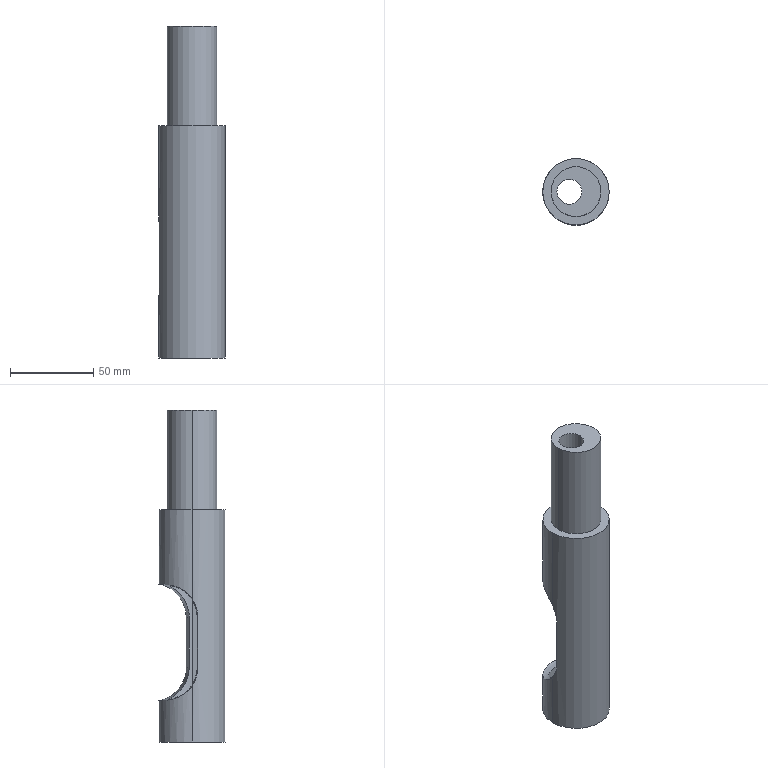Component | SolidWorks | 13EccentricSleeve-1 | 1 solid | 19 faces | box 40 x 40 x 200 mm | volume 119735 mm3 | cylinder 12 | plane 7 | commonest cylinder face diameters 40 x4 15 x2 16 x2 27.5 x2 30 x2
build123d program:
from build123d import *

# Parameters (mm, degrees)
SKETCH1_R               = 20
BOSS_EXTRUDE1_DEPTH     = 140
SKETCH2_R               = 15
BOSS_EXTRUDE2_DEPTH     = 60
SKETCH3_R               = 13.75
CUT_EXTRUDE1_DEPTH      = 100
SKETCH4_R               = 8
CUT_EXTRUDE2_DEPTH      = 80
SKETCH5_R               = 7.5
CUT_EXTRUDE3_DEPTH      = 183.209
CUT_EXTRUDE4_DEPTH      = 202.99
CUT_EXTRUDE4_DEPTH_BACK = 202.99


with BuildPart() as part:
    # Sketch1 → Boss-Extrude1 (new body)
    with BuildSketch(Plane(origin=(0, 0, 0), x_dir=(0, 0, -1), z_dir=(1, 0, 0))):
        Circle(SKETCH1_R)
    extrude(amount=BOSS_EXTRUDE1_DEPTH)

    # Sketch2 → Boss-Extrude2 (add)
    with BuildSketch(Plane(origin=(140, 0, 0), x_dir=(0, 0, -1), z_dir=(1, 0, 0))):
        Circle(SKETCH2_R)
    extrude(amount=BOSS_EXTRUDE2_DEPTH)

    # Sketch3 → Cut-Extrude1 (cut)
    with BuildSketch(Plane.ZY):
        with Locations((4, 0)):
            Circle(SKETCH3_R)
    extrude(amount=-CUT_EXTRUDE1_DEPTH, mode=Mode.SUBTRACT)

    # Sketch4 → Cut-Extrude2 (cut)
    with BuildSketch(Plane.ZY.offset(-100)):
        with Locations((4, 0)):
            Circle(SKETCH4_R)
    extrude(amount=-CUT_EXTRUDE2_DEPTH, mode=Mode.SUBTRACT)

    # Sketch5 → Cut-Extrude3 (cut, through all)
    with BuildSketch(Plane.ZY.offset(-180)):
        with Locations((4, 0)):
            Circle(SKETCH5_R)
    extrude(amount=-CUT_EXTRUDE3_DEPTH, mode=Mode.SUBTRACT)

    # Sketch8 → Cut-Extrude4 (cut, two sides: drawn at the far end of the back side and taken through both)
    with BuildSketch(Plane(origin=(0, 0, 0), x_dir=(-1, 0, 0), z_dir=(0, 0.1736, -0.9848)).offset(-CUT_EXTRUDE4_DEPTH_BACK)):
        with BuildLine():
            Line((-45, 0), (-75, 0))
            ThreePointArc((-75, 0), (-95, 20), (-75, 40))
            Line((-75, 40), (-45, 40))
            ThreePointArc((-45, 40), (-25, 20), (-45, 0))
        make_face()
    extrude(amount=CUT_EXTRUDE4_DEPTH + CUT_EXTRUDE4_DEPTH_BACK, mode=Mode.SUBTRACT)


solid = part.part

# Placed as in the assembly
solid = solid.moved(Location((37.957, -55.224, 190), (0, -90, 0)))
STEP:
#1=COLOUR_RGB('',0.7922,0.8196,0.9333);
#2=FILL_AREA_STYLE_COLOUR('',#1);
#3=FILL_AREA_STYLE('',(#2));
#4=SURFACE_STYLE_FILL_AREA(#3);
#5=SURFACE_SIDE_STYLE('',(#4));
#6=SURFACE_STYLE_USAGE(.BOTH.,#5);
#7=PRESENTATION_STYLE_ASSIGNMENT((#6));
#8=CARTESIAN_POINT('',(1.632,-2.174,15.354));
#9=VERTEX_POINT('',#8);
#10=CARTESIAN_POINT('',(1.042,-2.174,15.354));
#11=VERTEX_POINT('',#10);
#12=CARTESIAN_POINT('',(1.337,-2.174,15.354));
#13=DIRECTION('',(0.,-0.,-1.));
#14=DIRECTION('',(-1.,0.,0.));
#15=AXIS2_PLACEMENT_3D('',#12,#13,#14);
#16=CIRCLE('',#15,0.2953);
#17=EDGE_CURVE('',#9,#11,#16,.T.);
#18=ORIENTED_EDGE('',*,*,#17,.F.);
#19=CARTESIAN_POINT('',(1.632,-2.174,14.567));
#20=VERTEX_POINT('',#19);
#21=CARTESIAN_POINT('',(1.632,-2.174,15.354));
#22=DIRECTION('',(0.,-0.,-1.));
#23=VECTOR('',#22,39.37);
#24=LINE('',#21,#23);
#25=EDGE_CURVE('',#9,#20,#24,.T.);
#26=ORIENTED_EDGE('',*,*,#25,.T.);
#27=CARTESIAN_POINT('',(1.042,-2.174,14.567));
#28=VERTEX_POINT('',#27);
#29=CARTESIAN_POINT('',(1.337,-2.174,14.567));
#30=DIRECTION('',(0.,-0.,-1.));
#31=DIRECTION('',(-1.,0.,0.));
#32=AXIS2_PLACEMENT_3D('',#29,#30,#31);
#33=CIRCLE('',#32,0.2953);
#34=EDGE_CURVE('',#20,#28,#33,.T.);
#35=ORIENTED_EDGE('',*,*,#34,.T.);
#36=CARTESIAN_POINT('',(1.042,-2.174,15.354));
#37=DIRECTION('',(0.,-0.,-1.));
#38=VECTOR('',#37,39.37);
#39=LINE('',#36,#38);
#40=EDGE_CURVE('',#11,#28,#39,.T.);
#41=ORIENTED_EDGE('',*,*,#40,.F.);
#42=EDGE_LOOP('',(#18,#26,#35,#41));
#43=FACE_OUTER_BOUND('',#42,.T.);
#44=CARTESIAN_POINT('',(1.337,-2.174,15.354));
#45=DIRECTION('',(0.,-0.,-1.));
#46=DIRECTION('',(-1.,0.,0.));
#47=AXIS2_PLACEMENT_3D('',#44,#45,#46);
#48=CYLINDRICAL_SURFACE('',#47,0.2953);
#49=ADVANCED_FACE('',(#43),#48,.F.);
#50=CARTESIAN_POINT('',(1.652,-2.174,14.567));
#51=VERTEX_POINT('',#50);
#52=CARTESIAN_POINT('',(1.022,-2.174,14.567));
#53=VERTEX_POINT('',#52);
#54=CARTESIAN_POINT('',(1.337,-2.174,14.567));
#55=DIRECTION('',(0.,-0.,-1.));
#56=DIRECTION('',(1.,0.,0.));
#57=AXIS2_PLACEMENT_3D('',#54,#55,#56);
#58=CIRCLE('',#57,0.315);
#59=EDGE_CURVE('',#51,#53,#58,.T.);
#60=ORIENTED_EDGE('',*,*,#59,.F.);
#61=CARTESIAN_POINT('',(1.652,-2.174,11.417));
#62=VERTEX_POINT('',#61);
#63=CARTESIAN_POINT('',(1.652,-2.174,16.245));
#64=DIRECTION('',(0.,-0.,-1.));
#65=VECTOR('',#64,39.37);
#66=LINE('',#63,#65);
#67=EDGE_CURVE('',#51,#62,#66,.T.);
#68=ORIENTED_EDGE('',*,*,#67,.T.);
#69=CARTESIAN_POINT('',(1.022,-2.174,11.417));
#70=VERTEX_POINT('',#69);
#71=CARTESIAN_POINT('',(1.337,-2.174,11.417));
#72=DIRECTION('',(0.,-0.,-1.));
#73=DIRECTION('',(-1.,0.,0.));
#74=AXIS2_PLACEMENT_3D('',#71,#72,#73);
#75=CIRCLE('',#74,0.315);
#76=EDGE_CURVE('',#62,#70,#75,.T.);
#77=ORIENTED_EDGE('',*,*,#76,.T.);
#78=CARTESIAN_POINT('',(1.022,-2.174,16.245));
#79=DIRECTION('',(0.,-0.,-1.));
#80=VECTOR('',#79,39.37);
#81=LINE('',#78,#80);
#82=EDGE_CURVE('',#53,#70,#81,.T.);
#83=ORIENTED_EDGE('',*,*,#82,.F.);
#84=EDGE_LOOP('',(#60,#68,#77,#83));
#85=FACE_OUTER_BOUND('',#84,.T.);
#86=CARTESIAN_POINT('',(1.337,-2.174,16.245));
#87=DIRECTION('',(0.,-0.,-1.));
#88=DIRECTION('',(-1.,0.,0.));
#89=AXIS2_PLACEMENT_3D('',#86,#87,#88);
#90=CYLINDRICAL_SURFACE('',#89,0.315);
#91=ADVANCED_FACE('',(#85),#90,.F.);
#92=CARTESIAN_POINT('',(1.878,-2.174,11.417));
#93=VERTEX_POINT('',#92);
#94=CARTESIAN_POINT('',(0.7956,-2.174,11.417));
#95=VERTEX_POINT('',#94);
#96=CARTESIAN_POINT('',(1.337,-2.174,11.417));
#97=DIRECTION('',(0.,-0.,-1.));
#98=DIRECTION('',(-1.,0.,0.));
#99=AXIS2_PLACEMENT_3D('',#96,#97,#98);
#100=CIRCLE('',#99,0.5413);
#101=EDGE_CURVE('',#93,#95,#100,.T.);
#102=ORIENTED_EDGE('',*,*,#101,.F.);
#103=CARTESIAN_POINT('',(1.878,-2.174,7.48));
#104=VERTEX_POINT('',#103);
#105=CARTESIAN_POINT('',(1.878,-2.174,11.417));
#106=DIRECTION('',(0.,-0.,-1.));
#107=VECTOR('',#106,39.37);
#108=LINE('',#105,#107);
#109=EDGE_CURVE('',#93,#104,#108,.T.);
#110=ORIENTED_EDGE('',*,*,#109,.T.);
#111=CARTESIAN_POINT('',(0.7956,-2.174,7.48));
#112=VERTEX_POINT('',#111);
#113=CARTESIAN_POINT('',(1.337,-2.174,7.48));
#114=DIRECTION('',(0.,-0.,-1.));
#115=DIRECTION('',(-1.,0.,0.));
#116=AXIS2_PLACEMENT_3D('',#113,#114,#115);
#117=CIRCLE('',#116,0.5413);
#118=EDGE_CURVE('',#104,#112,#117,.T.);
#119=ORIENTED_EDGE('',*,*,#118,.T.);
#120=CARTESIAN_POINT('',(0.7956,-2.174,8.832));
#121=VERTEX_POINT('',#120);
#122=CARTESIAN_POINT('',(0.7956,-2.174,11.417));
#123=DIRECTION('',(0.,-0.,-1.));
#124=VECTOR('',#123,39.37);
#125=LINE('',#122,#124);
#126=EDGE_CURVE('',#121,#112,#125,.T.);
#127=ORIENTED_EDGE('',*,*,#126,.F.);
#128=CARTESIAN_POINT('',(0.8092,-2.295,9.252));
#129=VERTEX_POINT('',#128);
#130=CARTESIAN_POINT('',(0.7956,-2.174,8.832));
#131=CARTESIAN_POINT('',(0.7956,-2.194,8.863));
#132=CARTESIAN_POINT('',(0.7966,-2.211,8.895));
#133=CARTESIAN_POINT('',(0.7988,-2.234,8.946));
#134=CARTESIAN_POINT('',(0.7997,-2.241,8.963));
#135=CARTESIAN_POINT('',(0.8014,-2.254,8.998));
#136=CARTESIAN_POINT('',(0.8023,-2.259,9.015));
#137=CARTESIAN_POINT('',(0.8049,-2.275,9.068));
#138=CARTESIAN_POINT('',(0.8064,-2.282,9.104));
#139=CARTESIAN_POINT('',(0.8086,-2.292,9.178));
#140=CARTESIAN_POINT('',(0.8092,-2.295,9.215));
#141=CARTESIAN_POINT('',(0.8092,-2.295,9.252));
#142=B_SPLINE_CURVE_WITH_KNOTS('',3,(#130,#131,#132,#133,#134,#135,#136,#137,#138,#139,#140,#141),.UNSPECIFIED.,.F.,.F.,(4,2,2,2,2,4),(0.05482,0.05761,0.059,0.0604,0.06318,0.06597),.UNSPECIFIED.);
#143=EDGE_CURVE('',#121,#129,#142,.T.);
#144=ORIENTED_EDGE('',*,*,#143,.T.);
#145=CARTESIAN_POINT('',(0.8092,-2.295,10.433));
#146=VERTEX_POINT('',#145);
#147=CARTESIAN_POINT('',(0.8092,-2.295,11.417));
#148=DIRECTION('',(-0.,0.,1.));
#149=VECTOR('',#148,39.37);
#150=LINE('',#147,#149);
#151=EDGE_CURVE('',#129,#146,#150,.T.);
#152=ORIENTED_EDGE('',*,*,#151,.T.);
#153=CARTESIAN_POINT('',(0.7956,-2.174,10.853));
#154=VERTEX_POINT('',#153);
#155=CARTESIAN_POINT('',(0.8092,-2.295,10.433));
#156=CARTESIAN_POINT('',(0.8092,-2.295,10.47));
#157=CARTESIAN_POINT('',(0.8086,-2.292,10.507));
#158=CARTESIAN_POINT('',(0.8064,-2.282,10.58));
#159=CARTESIAN_POINT('',(0.8049,-2.275,10.616));
#160=CARTESIAN_POINT('',(0.8015,-2.255,10.687));
#161=CARTESIAN_POINT('',(0.7996,-2.242,10.722));
#162=CARTESIAN_POINT('',(0.7966,-2.211,10.79));
#163=CARTESIAN_POINT('',(0.7956,-2.194,10.822));
#164=CARTESIAN_POINT('',(0.7956,-2.174,10.853));
#165=B_SPLINE_CURVE_WITH_KNOTS('',3,(#155,#156,#157,#158,#159,#160,#161,#162,#163,#164),.UNSPECIFIED.,.F.,.F.,(4,2,2,2,4),(0.,0.002801,0.005603,0.008404,0.01121),.UNSPECIFIED.);
#166=EDGE_CURVE('',#146,#154,#165,.T.);
#167=ORIENTED_EDGE('',*,*,#166,.T.);
#168=CARTESIAN_POINT('',(0.7956,-2.174,11.417));
#169=DIRECTION('',(0.,-0.,-1.));
#170=VECTOR('',#169,39.37);
#171=LINE('',#168,#170);
#172=EDGE_CURVE('',#95,#154,#171,.T.);
#173=ORIENTED_EDGE('',*,*,#172,.F.);
#174=EDGE_LOOP('',(#102,#110,#119,#127,#144,#152,#167,#173));
#175=FACE_OUTER_BOUND('',#174,.T.);
#176=CARTESIAN_POINT('',(1.337,-2.174,11.417));
#177=DIRECTION('',(0.,-0.,-1.));
#178=DIRECTION('',(-1.,0.,0.));
#179=AXIS2_PLACEMENT_3D('',#176,#177,#178);
#180=CYLINDRICAL_SURFACE('',#179,0.5413);
#181=ADVANCED_FACE('',(#175),#180,.F.);
#182=CARTESIAN_POINT('',(2.085,-2.174,15.354));
#183=VERTEX_POINT('',#182);
#184=CARTESIAN_POINT('',(0.9038,-2.174,15.354));
#185=VERTEX_POINT('',#184);
#186=CARTESIAN_POINT('',(1.494,-2.174,15.354));
#187=DIRECTION('',(-0.,0.,1.));
#188=DIRECTION('',(1.,0.,0.));
#189=AXIS2_PLACEMENT_3D('',#186,#187,#188);
#190=CIRCLE('',#189,0.5906);
#191=EDGE_CURVE('',#183,#185,#190,.T.);
#192=ORIENTED_EDGE('',*,*,#191,.F.);
#193=CARTESIAN_POINT('',(2.085,-2.174,12.992));
#194=VERTEX_POINT('',#193);
#195=CARTESIAN_POINT('',(2.085,-2.174,15.354));
#196=DIRECTION('',(0.,-0.,-1.));
#197=VECTOR('',#196,39.37);
#198=LINE('',#195,#197);
#199=EDGE_CURVE('',#183,#194,#198,.T.);
#200=ORIENTED_EDGE('',*,*,#199,.T.);
#201=CARTESIAN_POINT('',(0.9038,-2.174,12.992));
#202=VERTEX_POINT('',#201);
#203=CARTESIAN_POINT('',(1.494,-2.174,12.992));
#204=DIRECTION('',(-0.,0.,1.));
#205=DIRECTION('',(1.,0.,0.));
#206=AXIS2_PLACEMENT_3D('',#203,#204,#205);
#207=CIRCLE('',#206,0.5906);
#208=EDGE_CURVE('',#194,#202,#207,.T.);
#209=ORIENTED_EDGE('',*,*,#208,.T.);
#210=CARTESIAN_POINT('',(0.9038,-2.174,15.354));
#211=DIRECTION('',(0.,-0.,-1.));
#212=VECTOR('',#211,39.37);
#213=LINE('',#210,#212);
#214=EDGE_CURVE('',#185,#202,#213,.T.);
#215=ORIENTED_EDGE('',*,*,#214,.F.);
#216=EDGE_LOOP('',(#192,#200,#209,#215));
#217=FACE_OUTER_BOUND('',#216,.T.);
#218=CARTESIAN_POINT('',(1.494,-2.174,15.354));
#219=DIRECTION('',(0.,-0.,-1.));
#220=DIRECTION('',(-1.,0.,0.));
#221=AXIS2_PLACEMENT_3D('',#218,#219,#220);
#222=CYLINDRICAL_SURFACE('',#221,0.5906);
#223=ADVANCED_FACE('',(#217),#222,.T.);
#224=CARTESIAN_POINT('',(2.282,-2.174,12.992));
#225=VERTEX_POINT('',#224);
#226=CARTESIAN_POINT('',(0.707,-2.174,12.992));
#227=VERTEX_POINT('',#226);
#228=CARTESIAN_POINT('',(1.494,-2.174,12.992));
#229=DIRECTION('',(-0.,0.,1.));
#230=DIRECTION('',(1.,0.,0.));
#231=AXIS2_PLACEMENT_3D('',#228,#229,#230);
#232=CIRCLE('',#231,0.7874);
#233=EDGE_CURVE('',#225,#227,#232,.T.);
#234=ORIENTED_EDGE('',*,*,#233,.F.);
#235=CARTESIAN_POINT('',(2.282,-2.174,7.48));
#236=VERTEX_POINT('',#235);
#237=CARTESIAN_POINT('',(2.282,-2.174,12.992));
#238=DIRECTION('',(0.,-0.,-1.));
#239=VECTOR('',#238,39.37);
#240=LINE('',#237,#239);
#241=EDGE_CURVE('',#225,#236,#240,.T.);
#242=ORIENTED_EDGE('',*,*,#241,.T.);
#243=CARTESIAN_POINT('',(0.707,-2.174,7.48));
#244=VERTEX_POINT('',#243);
#245=CARTESIAN_POINT('',(1.494,-2.174,7.48));
#246=DIRECTION('',(-0.,0.,1.));
#247=DIRECTION('',(1.,0.,0.));
#248=AXIS2_PLACEMENT_3D('',#245,#246,#247);
#249=CIRCLE('',#248,0.7874);
#250=EDGE_CURVE('',#236,#244,#249,.T.);
#251=ORIENTED_EDGE('',*,*,#250,.T.);
#252=CARTESIAN_POINT('',(0.707,-2.174,8.809));
#253=VERTEX_POINT('',#252);
#254=CARTESIAN_POINT('',(0.707,-2.174,12.992));
#255=DIRECTION('',(0.,-0.,-1.));
#256=VECTOR('',#255,39.37);
#257=LINE('',#254,#256);
#258=EDGE_CURVE('',#253,#244,#257,.T.);
#259=ORIENTED_EDGE('',*,*,#258,.F.);
#260=CARTESIAN_POINT('',(2.27,-2.037,9.252));
#261=VERTEX_POINT('',#260);
#262=CARTESIAN_POINT('',(0.707,-2.174,8.809));
#263=CARTESIAN_POINT('',(0.707,-2.166,8.796));
#264=CARTESIAN_POINT('',(0.7071,-2.157,8.784));
#265=CARTESIAN_POINT('',(0.7078,-2.138,8.76));
#266=CARTESIAN_POINT('',(0.7082,-2.128,8.749));
#267=CARTESIAN_POINT('',(0.7104,-2.098,8.715));
#268=CARTESIAN_POINT('',(0.7126,-2.077,8.694));
#269=CARTESIAN_POINT('',(0.7194,-2.033,8.655));
#270=CARTESIAN_POINT('',(0.7239,-2.01,8.636));
#271=CARTESIAN_POINT('',(0.7328,-1.974,8.611));
#272=CARTESIAN_POINT('',(0.7362,-1.961,8.603));
#273=CARTESIAN_POINT('',(0.7436,-1.936,8.588));
#274=CARTESIAN_POINT('',(0.7477,-1.924,8.58));
#275=CARTESIAN_POINT('',(0.7611,-1.886,8.56));
#276=CARTESIAN_POINT('',(0.7715,-1.861,8.548));
#277=CARTESIAN_POINT('',(0.7896,-1.823,8.532));
#278=CARTESIAN_POINT('',(0.796,-1.81,8.527));
#279=CARTESIAN_POINT('',(0.8097,-1.785,8.518));
#280=CARTESIAN_POINT('',(0.817,-1.772,8.514));
#281=CARTESIAN_POINT('',(0.8555,-1.71,8.494));
#282=CARTESIAN_POINT('',(0.892,-1.664,8.485));
#283=CARTESIAN_POINT('',(0.9448,-1.61,8.476));
#284=CARTESIAN_POINT('',(0.9558,-1.6,8.475));
#285=CARTESIAN_POINT('',(0.9781,-1.579,8.473));
#286=CARTESIAN_POINT('',(0.9895,-1.57,8.471));
#287=CARTESIAN_POINT('',(1.025,-1.542,8.469));
#288=CARTESIAN_POINT('',(1.049,-1.524,8.468));
#289=CARTESIAN_POINT('',(1.087,-1.5,8.466));
#290=CARTESIAN_POINT('',(1.1,-1.492,8.466));
#291=CARTESIAN_POINT('',(1.126,-1.478,8.465));
#292=CARTESIAN_POINT('',(1.14,-1.471,8.465));
#293=CARTESIAN_POINT('',(1.181,-1.451,8.465));
#294=CARTESIAN_POINT('',(1.208,-1.44,8.465));
#295=CARTESIAN_POINT('',(1.265,-1.42,8.465));
#296=CARTESIAN_POINT('',(1.294,-1.412,8.465));
#297=CARTESIAN_POINT('',(1.352,-1.399,8.465));
#298=CARTESIAN_POINT('',(1.382,-1.394,8.465));
#299=CARTESIAN_POINT('',(1.472,-1.385,8.465));
#300=CARTESIAN_POINT('',(1.532,-1.385,8.465));
#301=CARTESIAN_POINT('',(1.621,-1.397,8.466));
#302=CARTESIAN_POINT('',(1.651,-1.402,8.466));
#303=CARTESIAN_POINT('',(1.71,-1.416,8.468));
#304=CARTESIAN_POINT('',(1.738,-1.425,8.47));
#305=CARTESIAN_POINT('',(1.794,-1.445,8.474));
#306=CARTESIAN_POINT('',(1.822,-1.457,8.477));
#307=CARTESIAN_POINT('',(1.862,-1.477,8.482));
#308=CARTESIAN_POINT('',(1.875,-1.485,8.484));
#309=CARTESIAN_POINT('',(1.901,-1.5,8.489));
#310=CARTESIAN_POINT('',(1.913,-1.507,8.491));
#311=CARTESIAN_POINT('',(1.975,-1.548,8.505));
#312=CARTESIAN_POINT('',(2.019,-1.584,8.521));
#313=CARTESIAN_POINT('',(2.068,-1.635,8.549));
#314=CARTESIAN_POINT('',(2.078,-1.645,8.555));
#315=CARTESIAN_POINT('',(2.096,-1.665,8.568));
#316=CARTESIAN_POINT('',(2.104,-1.676,8.575));
#317=CARTESIAN_POINT('',(2.129,-1.707,8.597));
#318=CARTESIAN_POINT('',(2.143,-1.727,8.612));
#319=CARTESIAN_POINT('',(2.17,-1.769,8.647));
#320=CARTESIAN_POINT('',(2.182,-1.789,8.667));
#321=CARTESIAN_POINT('',(2.202,-1.828,8.708));
#322=CARTESIAN_POINT('',(2.211,-1.847,8.729));
#323=CARTESIAN_POINT('',(2.222,-1.874,8.764));
#324=CARTESIAN_POINT('',(2.226,-1.882,8.776));
#325=CARTESIAN_POINT('',(2.232,-1.899,8.8));
#326=CARTESIAN_POINT('',(2.235,-1.907,8.812));
#327=CARTESIAN_POINT('',(2.243,-1.931,8.85));
#328=CARTESIAN_POINT('',(2.248,-1.945,8.876));
#329=CARTESIAN_POINT('',(2.255,-1.971,8.93));
#330=CARTESIAN_POINT('',(2.258,-1.982,8.958));
#331=CARTESIAN_POINT('',(2.263,-2.002,9.015));
#332=CARTESIAN_POINT('',(2.265,-2.011,9.044));
#333=CARTESIAN_POINT('',(2.269,-2.031,9.132));
#334=CARTESIAN_POINT('',(2.27,-2.037,9.191));
#335=CARTESIAN_POINT('',(2.27,-2.037,9.252));
#336=B_SPLINE_CURVE_WITH_KNOTS('',3,(#262,#263,#264,#265,#266,#267,#268,#269,#270,#271,#272,#273,#274,#275,#276,#277,#278,#279,#280,#281,#282,#283,#284,#285,#286,#287,#288,#289,#290,#291,#292,#293,#294,#295,#296,#297,#298,#299,#300,#301,#302,#303,#304,#305,#306,#307,#308,#309,#310,#311,#312,#313,#314,#315,#316,#317,#318,#319,#320,#321,#322,#323,#324,#325,#326,#327,#328,#329,#330,#331,#332,#333,#334,#335),.UNSPECIFIED.,.F.,.F.,(4,2,2,2,2,2,2,2,2,2,2,2,2,2,2,2,2,2,2,2,2,2,2,2,2,2,2,2,2,2,2,2,2,2,2,2,4),(0.01193,0.01306,0.0142,0.01648,0.01875,0.01989,0.02103,0.0233,0.02444,0.02558,0.03013,0.03126,0.0324,0.03468,0.03581,0.03695,0.03923,0.0415,0.04378,0.04833,0.0506,0.05288,0.05515,0.05629,0.05743,0.06198,0.06311,0.06425,0.06652,0.0688,0.07107,0.07221,0.07335,0.07562,0.0779,0.08017,0.08472),.UNSPECIFIED.);
#337=EDGE_CURVE('',#253,#261,#336,.T.);
#338=ORIENTED_EDGE('',*,*,#337,.T.);
#339=CARTESIAN_POINT('',(2.27,-2.037,10.433));
#340=VERTEX_POINT('',#339);
#341=CARTESIAN_POINT('',(2.27,-2.037,12.992));
#342=DIRECTION('',(-0.,0.,1.));
#343=VECTOR('',#342,39.37);
#344=LINE('',#341,#343);
#345=EDGE_CURVE('',#261,#340,#344,.T.);
#346=ORIENTED_EDGE('',*,*,#345,.T.);
#347=CARTESIAN_POINT('',(0.707,-2.174,10.876));
#348=VERTEX_POINT('',#347);
#349=CARTESIAN_POINT('',(2.27,-2.037,10.433));
#350=CARTESIAN_POINT('',(2.27,-2.037,10.494));
#351=CARTESIAN_POINT('',(2.269,-2.031,10.553));
#352=CARTESIAN_POINT('',(2.265,-2.011,10.641));
#353=CARTESIAN_POINT('',(2.263,-2.002,10.67));
#354=CARTESIAN_POINT('',(2.258,-1.983,10.727));
#355=CARTESIAN_POINT('',(2.255,-1.971,10.754));
#356=CARTESIAN_POINT('',(2.248,-1.946,10.808));
#357=CARTESIAN_POINT('',(2.244,-1.932,10.834));
#358=CARTESIAN_POINT('',(2.236,-1.908,10.871));
#359=CARTESIAN_POINT('',(2.233,-1.9,10.884));
#360=CARTESIAN_POINT('',(2.226,-1.884,10.908));
#361=CARTESIAN_POINT('',(2.223,-1.875,10.92));
#362=CARTESIAN_POINT('',(2.204,-1.83,10.978));
#363=CARTESIAN_POINT('',(2.184,-1.791,11.018));
#364=CARTESIAN_POINT('',(2.151,-1.74,11.062));
#365=CARTESIAN_POINT('',(2.144,-1.73,11.07));
#366=CARTESIAN_POINT('',(2.13,-1.709,11.087));
#367=CARTESIAN_POINT('',(2.122,-1.698,11.094));
#368=CARTESIAN_POINT('',(2.097,-1.667,11.116));
#369=CARTESIAN_POINT('',(2.08,-1.647,11.129));
#370=CARTESIAN_POINT('',(2.041,-1.607,11.151));
#371=CARTESIAN_POINT('',(2.02,-1.587,11.161));
#372=CARTESIAN_POINT('',(1.987,-1.559,11.174));
#373=CARTESIAN_POINT('',(1.975,-1.55,11.178));
#374=CARTESIAN_POINT('',(1.952,-1.533,11.185));
#375=CARTESIAN_POINT('',(1.94,-1.525,11.188));
#376=CARTESIAN_POINT('',(1.903,-1.5,11.196));
#377=CARTESIAN_POINT('',(1.877,-1.485,11.201));
#378=CARTESIAN_POINT('',(1.837,-1.465,11.206));
#379=CARTESIAN_POINT('',(1.823,-1.459,11.208));
#380=CARTESIAN_POINT('',(1.796,-1.446,11.211));
#381=CARTESIAN_POINT('',(1.782,-1.441,11.212));
#382=CARTESIAN_POINT('',(1.739,-1.425,11.215));
#383=CARTESIAN_POINT('',(1.711,-1.416,11.217));
#384=CARTESIAN_POINT('',(1.667,-1.406,11.218));
#385=CARTESIAN_POINT('',(1.652,-1.403,11.219));
#386=CARTESIAN_POINT('',(1.623,-1.397,11.219));
#387=CARTESIAN_POINT('',(1.608,-1.395,11.219));
#388=CARTESIAN_POINT('',(1.533,-1.385,11.22));
#389=CARTESIAN_POINT('',(1.473,-1.385,11.22));
#390=CARTESIAN_POINT('',(1.398,-1.393,11.22));
#391=CARTESIAN_POINT('',(1.383,-1.395,11.22));
#392=CARTESIAN_POINT('',(1.353,-1.399,11.22));
#393=CARTESIAN_POINT('',(1.338,-1.402,11.22));
#394=CARTESIAN_POINT('',(1.294,-1.412,11.22));
#395=CARTESIAN_POINT('',(1.265,-1.42,11.22));
#396=CARTESIAN_POINT('',(1.209,-1.44,11.22));
#397=CARTESIAN_POINT('',(1.181,-1.451,11.22));
#398=CARTESIAN_POINT('',(1.14,-1.471,11.22));
#399=CARTESIAN_POINT('',(1.127,-1.478,11.22));
#400=CARTESIAN_POINT('',(1.101,-1.492,11.219));
#401=CARTESIAN_POINT('',(1.088,-1.5,11.219));
#402=CARTESIAN_POINT('',(1.024,-1.54,11.217));
#403=CARTESIAN_POINT('',(0.9773,-1.577,11.214));
#404=CARTESIAN_POINT('',(0.9247,-1.63,11.206));
#405=CARTESIAN_POINT('',(0.9145,-1.641,11.204));
#406=CARTESIAN_POINT('',(0.8946,-1.664,11.2));
#407=CARTESIAN_POINT('',(0.885,-1.675,11.197));
#408=CARTESIAN_POINT('',(0.8575,-1.71,11.189));
#409=CARTESIAN_POINT('',(0.8407,-1.734,11.183));
#410=CARTESIAN_POINT('',(0.8103,-1.783,11.168));
#411=CARTESIAN_POINT('',(0.7966,-1.808,11.159));
#412=CARTESIAN_POINT('',(0.7783,-1.846,11.143));
#413=CARTESIAN_POINT('',(0.7725,-1.859,11.138));
#414=CARTESIAN_POINT('',(0.7619,-1.885,11.125));
#415=CARTESIAN_POINT('',(0.757,-1.898,11.119));
#416=CARTESIAN_POINT('',(0.7435,-1.935,11.098));
#417=CARTESIAN_POINT('',(0.7362,-1.96,11.083));
#418=CARTESIAN_POINT('',(0.7272,-1.996,11.058));
#419=CARTESIAN_POINT('',(0.7245,-2.008,11.049));
#420=CARTESIAN_POINT('',(0.7199,-2.032,11.031));
#421=CARTESIAN_POINT('',(0.7178,-2.043,11.021));
#422=CARTESIAN_POINT('',(0.7092,-2.1,10.971));
#423=CARTESIAN_POINT('',(0.707,-2.14,10.926));
#424=CARTESIAN_POINT('',(0.707,-2.174,10.876));
#425=B_SPLINE_CURVE_WITH_KNOTS('',3,(#349,#350,#351,#352,#353,#354,#355,#356,#357,#358,#359,#360,#361,#362,#363,#364,#365,#366,#367,#368,#369,#370,#371,#372,#373,#374,#375,#376,#377,#378,#379,#380,#381,#382,#383,#384,#385,#386,#387,#388,#389,#390,#391,#392,#393,#394,#395,#396,#397,#398,#399,#400,#401,#402,#403,#404,#405,#406,#407,#408,#409,#410,#411,#412,#413,#414,#415,#416,#417,#418,#419,#420,#421,#422,#423,#424),.UNSPECIFIED.,.F.,.F.,(4,2,2,2,2,2,2,2,2,2,2,2,2,2,2,2,2,2,2,2,2,2,2,2,2,2,2,2,2,2,2,2,2,2,2,2,2,4),(0.,0.004553,0.00683,0.009107,0.01138,0.01252,0.01366,0.01821,0.01935,0.02049,0.02277,0.02504,0.02618,0.02732,0.0296,0.03074,0.03187,0.03415,0.03529,0.03643,0.04098,0.04212,0.04326,0.04553,0.04781,0.04895,0.05009,0.05464,0.05578,0.05692,0.05919,0.06147,0.06261,0.06375,0.06603,0.06716,0.0683,0.07286),.UNSPECIFIED.);
#426=EDGE_CURVE('',#340,#348,#425,.T.);
#427=ORIENTED_EDGE('',*,*,#426,.T.);
#428=CARTESIAN_POINT('',(0.707,-2.174,12.992));
#429=DIRECTION('',(0.,-0.,-1.));
#430=VECTOR('',#429,39.37);
#431=LINE('',#428,#430);
#432=EDGE_CURVE('',#227,#348,#431,.T.);
#433=ORIENTED_EDGE('',*,*,#432,.F.);
#434=EDGE_LOOP('',(#234,#242,#251,#259,#338,#346,#427,#433));
#435=FACE_OUTER_BOUND('',#434,.T.);
#436=CARTESIAN_POINT('',(1.494,-2.174,12.992));
#437=DIRECTION('',(0.,-0.,-1.));
#438=DIRECTION('',(-1.,0.,0.));
#439=AXIS2_PLACEMENT_3D('',#436,#437,#438);
#440=CYLINDRICAL_SURFACE('',#439,0.7874);
#441=ADVANCED_FACE('',(#435),#440,.T.);
#442=ORIENTED_EDGE('',*,*,#241,.F.);
#443=CARTESIAN_POINT('',(1.494,-2.174,12.992));
#444=DIRECTION('',(-0.,0.,1.));
#445=DIRECTION('',(1.,0.,0.));
#446=AXIS2_PLACEMENT_3D('',#443,#444,#445);
#447=CIRCLE('',#446,0.7874);
#448=EDGE_CURVE('',#227,#225,#447,.T.);
#449=ORIENTED_EDGE('',*,*,#448,.F.);
#450=ORIENTED_EDGE('',*,*,#432,.T.);
#451=CARTESIAN_POINT('',(0.7189,-2.311,10.433));
#452=VERTEX_POINT('',#451);
#453=CARTESIAN_POINT('',(0.707,-2.174,10.876));
#454=CARTESIAN_POINT('',(0.707,-2.185,10.86));
#455=CARTESIAN_POINT('',(0.7072,-2.196,10.844));
#456=CARTESIAN_POINT('',(0.708,-2.216,10.81));
#457=CARTESIAN_POINT('',(0.7086,-2.225,10.792));
#458=CARTESIAN_POINT('',(0.7105,-2.25,10.739));
#459=CARTESIAN_POINT('',(0.7121,-2.265,10.703));
#460=CARTESIAN_POINT('',(0.7151,-2.288,10.627));
#461=CARTESIAN_POINT('',(0.7165,-2.296,10.589));
#462=CARTESIAN_POINT('',(0.7184,-2.308,10.512));
#463=CARTESIAN_POINT('',(0.7189,-2.311,10.473));
#464=CARTESIAN_POINT('',(0.7189,-2.311,10.433));
#465=B_SPLINE_CURVE_WITH_KNOTS('',3,(#453,#454,#455,#456,#457,#458,#459,#460,#461,#462,#463,#464),.UNSPECIFIED.,.F.,.F.,(4,2,2,2,2,4),(0.07286,0.07434,0.07582,0.07879,0.08176,0.08472),.UNSPECIFIED.);
#466=EDGE_CURVE('',#348,#452,#465,.T.);
#467=ORIENTED_EDGE('',*,*,#466,.T.);
#468=CARTESIAN_POINT('',(0.7189,-2.311,9.252));
#469=VERTEX_POINT('',#468);
#470=CARTESIAN_POINT('',(0.7189,-2.311,12.992));
#471=DIRECTION('',(0.,-0.,-1.));
#472=VECTOR('',#471,39.37);
#473=LINE('',#470,#472);
#474=EDGE_CURVE('',#452,#469,#473,.T.);
#475=ORIENTED_EDGE('',*,*,#474,.T.);
#476=CARTESIAN_POINT('',(0.7189,-2.311,9.252));
#477=CARTESIAN_POINT('',(0.7189,-2.311,9.212));
#478=CARTESIAN_POINT('',(0.7184,-2.308,9.173));
#479=CARTESIAN_POINT('',(0.7165,-2.296,9.096));
#480=CARTESIAN_POINT('',(0.7151,-2.288,9.058));
#481=CARTESIAN_POINT('',(0.7129,-2.271,9.001));
#482=CARTESIAN_POINT('',(0.7121,-2.264,8.982));
#483=CARTESIAN_POINT('',(0.7106,-2.25,8.945));
#484=CARTESIAN_POINT('',(0.7098,-2.242,8.927));
#485=CARTESIAN_POINT('',(0.7079,-2.216,8.875));
#486=CARTESIAN_POINT('',(0.707,-2.197,8.841));
#487=CARTESIAN_POINT('',(0.707,-2.174,8.809));
#488=B_SPLINE_CURVE_WITH_KNOTS('',3,(#476,#477,#478,#479,#480,#481,#482,#483,#484,#485,#486,#487),.UNSPECIFIED.,.F.,.F.,(4,2,2,2,2,4),(0.,0.002982,0.005963,0.007454,0.008945,0.01193),.UNSPECIFIED.);
#489=EDGE_CURVE('',#469,#253,#488,.T.);
#490=ORIENTED_EDGE('',*,*,#489,.T.);
#491=ORIENTED_EDGE('',*,*,#258,.T.);
#492=CARTESIAN_POINT('',(1.494,-2.174,7.48));
#493=DIRECTION('',(-0.,0.,1.));
#494=DIRECTION('',(1.,0.,0.));
#495=AXIS2_PLACEMENT_3D('',#492,#493,#494);
#496=CIRCLE('',#495,0.7874);
#497=EDGE_CURVE('',#244,#236,#496,.T.);
#498=ORIENTED_EDGE('',*,*,#497,.T.);
#499=EDGE_LOOP('',(#442,#449,#450,#467,#475,#490,#491,#498));
#500=FACE_OUTER_BOUND('',#499,.T.);
#501=CARTESIAN_POINT('',(1.494,-2.174,12.992));
#502=DIRECTION('',(0.,-0.,-1.));
#503=DIRECTION('',(-1.,0.,0.));
#504=AXIS2_PLACEMENT_3D('',#501,#502,#503);
#505=CYLINDRICAL_SURFACE('',#504,0.7874);
#506=ADVANCED_FACE('',(#500),#505,.T.);
#507=CARTESIAN_POINT('',(1.494,-2.174,12.992));
#508=DIRECTION('',(-0.,0.,1.));
#509=DIRECTION('',(1.,0.,0.));
#510=AXIS2_PLACEMENT_3D('',#507,#508,#509);
#511=CIRCLE('',#510,0.5906);
#512=EDGE_CURVE('',#202,#194,#511,.T.);
#513=ORIENTED_EDGE('',*,*,#512,.F.);
#514=ORIENTED_EDGE('',*,*,#208,.F.);
#515=EDGE_LOOP('',(#513,#514));
#516=FACE_BOUND('',#515,.T.);
#517=ORIENTED_EDGE('',*,*,#448,.T.);
#518=ORIENTED_EDGE('',*,*,#233,.T.);
#519=EDGE_LOOP('',(#517,#518));
#520=FACE_OUTER_BOUND('',#519,.T.);
#521=CARTESIAN_POINT('',(1.494,-2.174,12.992));
#522=DIRECTION('',(-0.,0.,1.));
#523=DIRECTION('',(1.,0.,0.));
#524=AXIS2_PLACEMENT_3D('',#521,#522,#523);
#525=PLANE('',#524);
#526=ADVANCED_FACE('',(#516,#520),#525,.T.);
#527=CARTESIAN_POINT('',(1.337,-2.174,7.48));
#528=DIRECTION('',(0.,-0.,-1.));
#529=DIRECTION('',(-1.,0.,0.));
#530=AXIS2_PLACEMENT_3D('',#527,#528,#529);
#531=CIRCLE('',#530,0.5413);
#532=EDGE_CURVE('',#112,#104,#531,.T.);
#533=ORIENTED_EDGE('',*,*,#532,.F.);
#534=ORIENTED_EDGE('',*,*,#118,.F.);
#535=EDGE_LOOP('',(#533,#534));
#536=FACE_BOUND('',#535,.T.);
#537=ORIENTED_EDGE('',*,*,#497,.F.);
#538=ORIENTED_EDGE('',*,*,#250,.F.);
#539=EDGE_LOOP('',(#537,#538));
#540=FACE_OUTER_BOUND('',#539,.T.);
#541=CARTESIAN_POINT('',(1.494,-2.174,7.48));
#542=DIRECTION('',(-0.,0.,1.));
#543=DIRECTION('',(1.,0.,0.));
#544=AXIS2_PLACEMENT_3D('',#541,#542,#543);
#545=PLANE('',#544);
#546=ADVANCED_FACE('',(#536,#540),#545,.F.);
#547=ORIENTED_EDGE('',*,*,#199,.F.);
#548=CARTESIAN_POINT('',(1.494,-2.174,15.354));
#549=DIRECTION('',(-0.,0.,1.));
#550=DIRECTION('',(1.,0.,0.));
#551=AXIS2_PLACEMENT_3D('',#548,#549,#550);
#552=CIRCLE('',#551,0.5906);
#553=EDGE_CURVE('',#185,#183,#552,.T.);
#554=ORIENTED_EDGE('',*,*,#553,.F.);
#555=ORIENTED_EDGE('',*,*,#214,.T.);
#556=ORIENTED_EDGE('',*,*,#512,.T.);
#557=EDGE_LOOP('',(#547,#554,#555,#556));
#558=FACE_OUTER_BOUND('',#557,.T.);
#559=CARTESIAN_POINT('',(1.494,-2.174,15.354));
#560=DIRECTION('',(0.,-0.,-1.));
#561=DIRECTION('',(-1.,0.,0.));
#562=AXIS2_PLACEMENT_3D('',#559,#560,#561);
#563=CYLINDRICAL_SURFACE('',#562,0.5906);
#564=ADVANCED_FACE('',(#558),#563,.T.);
#565=CARTESIAN_POINT('',(1.337,-2.174,15.354));
#566=DIRECTION('',(0.,-0.,-1.));
#567=DIRECTION('',(-1.,0.,0.));
#568=AXIS2_PLACEMENT_3D('',#565,#566,#567);
#569=CIRCLE('',#568,0.2953);
#570=EDGE_CURVE('',#11,#9,#569,.T.);
#571=ORIENTED_EDGE('',*,*,#570,.T.);
#572=ORIENTED_EDGE('',*,*,#17,.T.);
#573=EDGE_LOOP('',(#571,#572));
#574=FACE_BOUND('',#573,.T.);
#575=ORIENTED_EDGE('',*,*,#553,.T.);
#576=ORIENTED_EDGE('',*,*,#191,.T.);
#577=EDGE_LOOP('',(#575,#576));
#578=FACE_OUTER_BOUND('',#577,.T.);
#579=CARTESIAN_POINT('',(1.494,-2.174,15.354));
#580=DIRECTION('',(-0.,0.,1.));
#581=DIRECTION('',(1.,0.,0.));
#582=AXIS2_PLACEMENT_3D('',#579,#580,#581);
#583=PLANE('',#582);
#584=ADVANCED_FACE('',(#574,#578),#583,.T.);
#585=ORIENTED_EDGE('',*,*,#109,.F.);
#586=CARTESIAN_POINT('',(1.337,-2.174,11.417));
#587=DIRECTION('',(0.,-0.,-1.));
#588=DIRECTION('',(-1.,0.,0.));
#589=AXIS2_PLACEMENT_3D('',#586,#587,#588);
#590=CIRCLE('',#589,0.5413);
#591=EDGE_CURVE('',#95,#93,#590,.T.);
#592=ORIENTED_EDGE('',*,*,#591,.F.);
#593=ORIENTED_EDGE('',*,*,#172,.T.);
#594=CARTESIAN_POINT('',(1.874,-2.107,10.433));
#595=VERTEX_POINT('',#594);
#596=CARTESIAN_POINT('',(0.7956,-2.174,10.853));
#597=CARTESIAN_POINT('',(0.7956,-2.162,10.872));
#598=CARTESIAN_POINT('',(0.796,-2.149,10.89));
#599=CARTESIAN_POINT('',(0.798,-2.121,10.926));
#600=CARTESIAN_POINT('',(0.7996,-2.106,10.944));
#601=CARTESIAN_POINT('',(0.8068,-2.06,10.993));
#602=CARTESIAN_POINT('',(0.8147,-2.027,11.022));
#603=CARTESIAN_POINT('',(0.8306,-1.982,11.055));
#604=CARTESIAN_POINT('',(0.8341,-1.973,11.061));
#605=CARTESIAN_POINT('',(0.8415,-1.956,11.073));
#606=CARTESIAN_POINT('',(0.8456,-1.947,11.079));
#607=CARTESIAN_POINT('',(0.8585,-1.92,11.095));
#608=CARTESIAN_POINT('',(0.8683,-1.902,11.105));
#609=CARTESIAN_POINT('',(0.885,-1.876,11.118));
#610=CARTESIAN_POINT('',(0.8908,-1.867,11.123));
#611=CARTESIAN_POINT('',(0.9032,-1.85,11.131));
#612=CARTESIAN_POINT('',(0.9098,-1.841,11.134));
#613=CARTESIAN_POINT('',(0.9303,-1.816,11.145));
#614=CARTESIAN_POINT('',(0.9451,-1.8,11.151));
#615=CARTESIAN_POINT('',(0.9767,-1.769,11.162));
#616=CARTESIAN_POINT('',(0.9936,-1.755,11.166));
#617=CARTESIAN_POINT('',(1.021,-1.735,11.172));
#618=CARTESIAN_POINT('',(1.03,-1.728,11.174));
#619=CARTESIAN_POINT('',(1.049,-1.716,11.177));
#620=CARTESIAN_POINT('',(1.058,-1.71,11.178));
#621=CARTESIAN_POINT('',(1.088,-1.693,11.182));
#622=CARTESIAN_POINT('',(1.108,-1.683,11.184));
#623=CARTESIAN_POINT('',(1.139,-1.67,11.186));
#624=CARTESIAN_POINT('',(1.15,-1.666,11.187));
#625=CARTESIAN_POINT('',(1.171,-1.659,11.188));
#626=CARTESIAN_POINT('',(1.182,-1.655,11.188));
#627=CARTESIAN_POINT('',(1.237,-1.64,11.19));
#628=CARTESIAN_POINT('',(1.282,-1.634,11.19));
#629=CARTESIAN_POINT('',(1.339,-1.633,11.187));
#630=CARTESIAN_POINT('',(1.35,-1.633,11.186));
#631=CARTESIAN_POINT('',(1.373,-1.634,11.185));
#632=CARTESIAN_POINT('',(1.384,-1.635,11.184));
#633=CARTESIAN_POINT('',(1.418,-1.638,11.181));
#634=CARTESIAN_POINT('',(1.44,-1.642,11.178));
#635=CARTESIAN_POINT('',(1.473,-1.65,11.174));
#636=CARTESIAN_POINT('',(1.484,-1.653,11.172));
#637=CARTESIAN_POINT('',(1.505,-1.659,11.168));
#638=CARTESIAN_POINT('',(1.516,-1.663,11.166));
#639=CARTESIAN_POINT('',(1.547,-1.675,11.159));
#640=CARTESIAN_POINT('',(1.567,-1.684,11.154));
#641=CARTESIAN_POINT('',(1.606,-1.704,11.142));
#642=CARTESIAN_POINT('',(1.624,-1.715,11.135));
#643=CARTESIAN_POINT('',(1.651,-1.733,11.123));
#644=CARTESIAN_POINT('',(1.659,-1.739,11.118));
#645=CARTESIAN_POINT('',(1.676,-1.752,11.109));
#646=CARTESIAN_POINT('',(1.684,-1.759,11.105));
#647=CARTESIAN_POINT('',(1.707,-1.779,11.09));
#648=CARTESIAN_POINT('',(1.721,-1.792,11.079));
#649=CARTESIAN_POINT('',(1.741,-1.814,11.061));
#650=CARTESIAN_POINT('',(1.747,-1.821,11.055));
#651=CARTESIAN_POINT('',(1.759,-1.835,11.042));
#652=CARTESIAN_POINT('',(1.765,-1.843,11.035));
#653=CARTESIAN_POINT('',(1.792,-1.879,11.));
#654=CARTESIAN_POINT('',(1.809,-1.907,10.969));
#655=CARTESIAN_POINT('',(1.828,-1.947,10.917));
#656=CARTESIAN_POINT('',(1.834,-1.96,10.899));
#657=CARTESIAN_POINT('',(1.844,-1.984,10.862));
#658=CARTESIAN_POINT('',(1.848,-1.995,10.843));
#659=CARTESIAN_POINT('',(1.855,-2.017,10.804));
#660=CARTESIAN_POINT('',(1.858,-2.027,10.784));
#661=CARTESIAN_POINT('',(1.863,-2.045,10.743));
#662=CARTESIAN_POINT('',(1.865,-2.054,10.721));
#663=CARTESIAN_POINT('',(1.87,-2.076,10.657));
#664=CARTESIAN_POINT('',(1.871,-2.088,10.614));
#665=CARTESIAN_POINT('',(1.874,-2.103,10.524));
#666=CARTESIAN_POINT('',(1.874,-2.107,10.479));
#667=CARTESIAN_POINT('',(1.874,-2.107,10.433));
#668=B_SPLINE_CURVE_WITH_KNOTS('',3,(#596,#597,#598,#599,#600,#601,#602,#603,#604,#605,#606,#607,#608,#609,#610,#611,#612,#613,#614,#615,#616,#617,#618,#619,#620,#621,#622,#623,#624,#625,#626,#627,#628,#629,#630,#631,#632,#633,#634,#635,#636,#637,#638,#639,#640,#641,#642,#643,#644,#645,#646,#647,#648,#649,#650,#651,#652,#653,#654,#655,#656,#657,#658,#659,#660,#661,#662,#663,#664,#665,#666,#667),.UNSPECIFIED.,.F.,.F.,(4,2,2,2,2,2,2,2,2,2,2,2,2,2,2,2,2,2,2,2,2,2,2,2,2,2,2,2,2,2,2,2,2,2,2,4),(0.01121,0.01292,0.01463,0.01805,0.01891,0.01976,0.02147,0.02233,0.02318,0.0249,0.02661,0.02746,0.02832,0.03003,0.03089,0.03174,0.03516,0.03602,0.03688,0.03859,0.03944,0.0403,0.04201,0.04372,0.04458,0.04543,0.04714,0.048,0.04886,0.05228,0.05399,0.0557,0.05741,0.05912,0.06255,0.06597),.UNSPECIFIED.);
#669=EDGE_CURVE('',#154,#595,#668,.T.);
#670=ORIENTED_EDGE('',*,*,#669,.T.);
#671=CARTESIAN_POINT('',(1.874,-2.107,9.252));
#672=VERTEX_POINT('',#671);
#673=CARTESIAN_POINT('',(1.874,-2.107,11.417));
#674=DIRECTION('',(0.,-0.,-1.));
#675=VECTOR('',#674,39.37);
#676=LINE('',#673,#675);
#677=EDGE_CURVE('',#595,#672,#676,.T.);
#678=ORIENTED_EDGE('',*,*,#677,.T.);
#679=CARTESIAN_POINT('',(1.874,-2.107,9.252));
#680=CARTESIAN_POINT('',(1.874,-2.107,9.206));
#681=CARTESIAN_POINT('',(1.874,-2.103,9.161));
#682=CARTESIAN_POINT('',(1.871,-2.088,9.073));
#683=CARTESIAN_POINT('',(1.87,-2.077,9.029));
#684=CARTESIAN_POINT('',(1.865,-2.054,8.965));
#685=CARTESIAN_POINT('',(1.863,-2.046,8.944));
#686=CARTESIAN_POINT('',(1.858,-2.027,8.903));
#687=CARTESIAN_POINT('',(1.855,-2.018,8.883));
#688=CARTESIAN_POINT('',(1.845,-1.986,8.824));
#689=CARTESIAN_POINT('',(1.836,-1.961,8.787));
#690=CARTESIAN_POINT('',(1.809,-1.908,8.718));
#691=CARTESIAN_POINT('',(1.793,-1.88,8.686));
#692=CARTESIAN_POINT('',(1.766,-1.844,8.651));
#693=CARTESIAN_POINT('',(1.76,-1.837,8.645));
#694=CARTESIAN_POINT('',(1.748,-1.822,8.632));
#695=CARTESIAN_POINT('',(1.742,-1.815,8.625));
#696=CARTESIAN_POINT('',(1.723,-1.794,8.607));
#697=CARTESIAN_POINT('',(1.708,-1.78,8.596));
#698=CARTESIAN_POINT('',(1.678,-1.753,8.576));
#699=CARTESIAN_POINT('',(1.662,-1.741,8.567));
#700=CARTESIAN_POINT('',(1.635,-1.722,8.555));
#701=CARTESIAN_POINT('',(1.626,-1.717,8.551));
#702=CARTESIAN_POINT('',(1.608,-1.705,8.544));
#703=CARTESIAN_POINT('',(1.598,-1.7,8.541));
#704=CARTESIAN_POINT('',(1.569,-1.685,8.532));
#705=CARTESIAN_POINT('',(1.549,-1.676,8.526));
#706=CARTESIAN_POINT('',(1.518,-1.664,8.519));
#707=CARTESIAN_POINT('',(1.507,-1.66,8.517));
#708=CARTESIAN_POINT('',(1.486,-1.654,8.513));
#709=CARTESIAN_POINT('',(1.475,-1.651,8.512));
#710=CARTESIAN_POINT('',(1.42,-1.637,8.504));
#711=CARTESIAN_POINT('',(1.375,-1.632,8.5));
#712=CARTESIAN_POINT('',(1.318,-1.633,8.497));
#713=CARTESIAN_POINT('',(1.307,-1.634,8.497));
#714=CARTESIAN_POINT('',(1.284,-1.635,8.496));
#715=CARTESIAN_POINT('',(1.273,-1.637,8.496));
#716=CARTESIAN_POINT('',(1.239,-1.641,8.495));
#717=CARTESIAN_POINT('',(1.217,-1.646,8.496));
#718=CARTESIAN_POINT('',(1.184,-1.655,8.497));
#719=CARTESIAN_POINT('',(1.173,-1.658,8.497));
#720=CARTESIAN_POINT('',(1.151,-1.665,8.498));
#721=CARTESIAN_POINT('',(1.141,-1.67,8.499));
#722=CARTESIAN_POINT('',(1.109,-1.683,8.501));
#723=CARTESIAN_POINT('',(1.089,-1.692,8.503));
#724=CARTESIAN_POINT('',(1.05,-1.715,8.508));
#725=CARTESIAN_POINT('',(1.031,-1.727,8.511));
#726=CARTESIAN_POINT('',(1.004,-1.747,8.517));
#727=CARTESIAN_POINT('',(0.9952,-1.754,8.519));
#728=CARTESIAN_POINT('',(0.9781,-1.769,8.523));
#729=CARTESIAN_POINT('',(0.9699,-1.776,8.526));
#730=CARTESIAN_POINT('',(0.946,-1.799,8.534));
#731=CARTESIAN_POINT('',(0.9313,-1.815,8.54));
#732=CARTESIAN_POINT('',(0.9108,-1.84,8.55));
#733=CARTESIAN_POINT('',(0.9043,-1.849,8.554));
#734=CARTESIAN_POINT('',(0.8918,-1.866,8.562));
#735=CARTESIAN_POINT('',(0.8858,-1.875,8.566));
#736=CARTESIAN_POINT('',(0.8576,-1.919,8.589));
#737=CARTESIAN_POINT('',(0.8405,-1.955,8.61));
#738=CARTESIAN_POINT('',(0.8245,-1.999,8.643));
#739=CARTESIAN_POINT('',(0.8216,-2.008,8.649));
#740=CARTESIAN_POINT('',(0.8164,-2.025,8.663));
#741=CARTESIAN_POINT('',(0.814,-2.034,8.67));
#742=CARTESIAN_POINT('',(0.8077,-2.059,8.693));
#743=CARTESIAN_POINT('',(0.8045,-2.075,8.708));
#744=CARTESIAN_POINT('',(0.7996,-2.106,8.741));
#745=CARTESIAN_POINT('',(0.798,-2.121,8.759));
#746=CARTESIAN_POINT('',(0.796,-2.149,8.794));
#747=CARTESIAN_POINT('',(0.7956,-2.162,8.813));
#748=CARTESIAN_POINT('',(0.7956,-2.174,8.832));
#749=B_SPLINE_CURVE_WITH_KNOTS('',3,(#679,#680,#681,#682,#683,#684,#685,#686,#687,#688,#689,#690,#691,#692,#693,#694,#695,#696,#697,#698,#699,#700,#701,#702,#703,#704,#705,#706,#707,#708,#709,#710,#711,#712,#713,#714,#715,#716,#717,#718,#719,#720,#721,#722,#723,#724,#725,#726,#727,#728,#729,#730,#731,#732,#733,#734,#735,#736,#737,#738,#739,#740,#741,#742,#743,#744,#745,#746,#747,#748),.UNSPECIFIED.,.F.,.F.,(4,2,2,2,2,2,2,2,2,2,2,2,2,2,2,2,2,2,2,2,2,2,2,2,2,2,2,2,2,2,2,2,2,2,4),(0.,0.003426,0.006853,0.008566,0.01028,0.01371,0.01713,0.01799,0.01885,0.02056,0.02227,0.02313,0.02398,0.0257,0.02655,0.02741,0.03084,0.03169,0.03255,0.03426,0.03512,0.03598,0.03769,0.0394,0.04026,0.04112,0.04283,0.04369,0.04454,0.04797,0.04883,0.04968,0.0514,0.05311,0.05482),.UNSPECIFIED.);
#750=EDGE_CURVE('',#672,#121,#749,.T.);
#751=ORIENTED_EDGE('',*,*,#750,.T.);
#752=ORIENTED_EDGE('',*,*,#126,.T.);
#753=ORIENTED_EDGE('',*,*,#532,.T.);
#754=EDGE_LOOP('',(#585,#592,#593,#670,#678,#751,#752,#753));
#755=FACE_OUTER_BOUND('',#754,.T.);
#756=CARTESIAN_POINT('',(1.337,-2.174,11.417));
#757=DIRECTION('',(0.,-0.,-1.));
#758=DIRECTION('',(-1.,0.,0.));
#759=AXIS2_PLACEMENT_3D('',#756,#757,#758);
#760=CYLINDRICAL_SURFACE('',#759,0.5413);
#761=ADVANCED_FACE('',(#755),#760,.F.);
#762=CARTESIAN_POINT('',(1.337,-2.174,11.417));
#763=DIRECTION('',(0.,-0.,-1.));
#764=DIRECTION('',(-1.,0.,0.));
#765=AXIS2_PLACEMENT_3D('',#762,#763,#764);
#766=CIRCLE('',#765,0.315);
#767=EDGE_CURVE('',#70,#62,#766,.T.);
#768=ORIENTED_EDGE('',*,*,#767,.F.);
#769=ORIENTED_EDGE('',*,*,#76,.F.);
#770=EDGE_LOOP('',(#768,#769));
#771=FACE_BOUND('',#770,.T.);
#772=ORIENTED_EDGE('',*,*,#591,.T.);
#773=ORIENTED_EDGE('',*,*,#101,.T.);
#774=EDGE_LOOP('',(#772,#773));
#775=FACE_OUTER_BOUND('',#774,.T.);
#776=CARTESIAN_POINT('',(1.337,-2.174,11.417));
#777=DIRECTION('',(0.,-0.,-1.));
#778=DIRECTION('',(-1.,-0.,-0.));
#779=AXIS2_PLACEMENT_3D('',#776,#777,#778);
#780=PLANE('',#779);
#781=ADVANCED_FACE('',(#771,#775),#780,.T.);
#782=CARTESIAN_POINT('',(1.337,-2.174,14.567));
#783=DIRECTION('',(0.,-0.,-1.));
#784=DIRECTION('',(-1.,0.,0.));
#785=AXIS2_PLACEMENT_3D('',#782,#783,#784);
#786=CIRCLE('',#785,0.2953);
#787=EDGE_CURVE('',#28,#20,#786,.T.);
#788=ORIENTED_EDGE('',*,*,#787,.F.);
#789=ORIENTED_EDGE('',*,*,#34,.F.);
#790=EDGE_LOOP('',(#788,#789));
#791=FACE_BOUND('',#790,.T.);
#792=CARTESIAN_POINT('',(1.337,-2.174,14.567));
#793=DIRECTION('',(0.,-0.,-1.));
#794=DIRECTION('',(1.,0.,0.));
#795=AXIS2_PLACEMENT_3D('',#792,#793,#794);
#796=CIRCLE('',#795,0.315);
#797=EDGE_CURVE('',#53,#51,#796,.T.);
#798=ORIENTED_EDGE('',*,*,#797,.T.);
#799=ORIENTED_EDGE('',*,*,#59,.T.);
#800=EDGE_LOOP('',(#798,#799));
#801=FACE_OUTER_BOUND('',#800,.T.);
#802=CARTESIAN_POINT('',(1.494,-2.174,14.567));
#803=DIRECTION('',(-0.,0.,1.));
#804=DIRECTION('',(1.,0.,0.));
#805=AXIS2_PLACEMENT_3D('',#802,#803,#804);
#806=PLANE('',#805);
#807=ADVANCED_FACE('',(#791,#801),#806,.F.);
#808=ORIENTED_EDGE('',*,*,#67,.F.);
#809=ORIENTED_EDGE('',*,*,#797,.F.);
#810=ORIENTED_EDGE('',*,*,#82,.T.);
#811=ORIENTED_EDGE('',*,*,#767,.T.);
#812=EDGE_LOOP('',(#808,#809,#810,#811));
#813=FACE_OUTER_BOUND('',#812,.T.);
#814=CARTESIAN_POINT('',(1.337,-2.174,16.245));
#815=DIRECTION('',(0.,-0.,-1.));
#816=DIRECTION('',(-1.,0.,0.));
#817=AXIS2_PLACEMENT_3D('',#814,#815,#816);
#818=CYLINDRICAL_SURFACE('',#817,0.315);
#819=ADVANCED_FACE('',(#813),#818,.F.);
#820=ORIENTED_EDGE('',*,*,#25,.F.);
#821=ORIENTED_EDGE('',*,*,#570,.F.);
#822=ORIENTED_EDGE('',*,*,#40,.T.);
#823=ORIENTED_EDGE('',*,*,#787,.T.);
#824=EDGE_LOOP('',(#820,#821,#822,#823));
#825=FACE_OUTER_BOUND('',#824,.T.);
#826=CARTESIAN_POINT('',(1.337,-2.174,15.354));
#827=DIRECTION('',(0.,-0.,-1.));
#828=DIRECTION('',(-1.,0.,0.));
#829=AXIS2_PLACEMENT_3D('',#826,#827,#828);
#830=CYLINDRICAL_SURFACE('',#829,0.2953);
#831=ADVANCED_FACE('',(#825),#830,.F.);
#832=CARTESIAN_POINT('',(0.5961,-2.333,9.252));
#833=DIRECTION('',(0.9848,0.1736,0.));
#834=VECTOR('',#833,39.37);
#835=LINE('',#832,#834);
#836=EDGE_CURVE('',#469,#129,#835,.T.);
#837=ORIENTED_EDGE('',*,*,#836,.T.);
#838=ORIENTED_EDGE('',*,*,#143,.F.);
#839=ORIENTED_EDGE('',*,*,#750,.F.);
#840=CARTESIAN_POINT('',(0.5961,-2.333,9.252));
#841=DIRECTION('',(0.9848,0.1736,0.));
#842=VECTOR('',#841,39.37);
#843=LINE('',#840,#842);
#844=EDGE_CURVE('',#672,#261,#843,.T.);
#845=ORIENTED_EDGE('',*,*,#844,.T.);
#846=ORIENTED_EDGE('',*,*,#337,.F.);
#847=ORIENTED_EDGE('',*,*,#489,.F.);
#848=EDGE_LOOP('',(#837,#838,#839,#845,#846,#847));
#849=FACE_OUTER_BOUND('',#848,.T.);
#850=CARTESIAN_POINT('',(0.4593,-1.557,9.252));
#851=DIRECTION('',(0.9848,0.1736,0.));
#852=DIRECTION('',(-0.1736,0.9848,0.));
#853=AXIS2_PLACEMENT_3D('',#850,#851,#852);
#854=CYLINDRICAL_SURFACE('',#853,0.7874);
#855=ADVANCED_FACE('',(#849),#854,.F.);
#856=CARTESIAN_POINT('',(0.5961,-2.333,10.433));
#857=DIRECTION('',(0.9848,0.1736,0.));
#858=VECTOR('',#857,39.37);
#859=LINE('',#856,#858);
#860=EDGE_CURVE('',#452,#146,#859,.T.);
#861=ORIENTED_EDGE('',*,*,#860,.T.);
#862=ORIENTED_EDGE('',*,*,#151,.F.);
#863=ORIENTED_EDGE('',*,*,#836,.F.);
#864=ORIENTED_EDGE('',*,*,#474,.F.);
#865=EDGE_LOOP('',(#861,#862,#863,#864));
#866=FACE_OUTER_BOUND('',#865,.T.);
#867=CARTESIAN_POINT('',(0.5961,-2.333,9.252));
#868=DIRECTION('',(0.1736,-0.9848,-0.));
#869=DIRECTION('',(0.9848,0.1736,0.));
#870=AXIS2_PLACEMENT_3D('',#867,#868,#869);
#871=PLANE('',#870);
#872=ADVANCED_FACE('',(#866),#871,.F.);
#873=ORIENTED_EDGE('',*,*,#844,.F.);
#874=ORIENTED_EDGE('',*,*,#677,.F.);
#875=CARTESIAN_POINT('',(0.5961,-2.333,10.433));
#876=DIRECTION('',(0.9848,0.1736,0.));
#877=VECTOR('',#876,39.37);
#878=LINE('',#875,#877);
#879=EDGE_CURVE('',#595,#340,#878,.T.);
#880=ORIENTED_EDGE('',*,*,#879,.T.);
#881=ORIENTED_EDGE('',*,*,#345,.F.);
#882=EDGE_LOOP('',(#873,#874,#880,#881));
#883=FACE_OUTER_BOUND('',#882,.T.);
#884=CARTESIAN_POINT('',(0.5961,-2.333,9.252));
#885=DIRECTION('',(0.1736,-0.9848,-0.));
#886=DIRECTION('',(0.9848,0.1736,0.));
#887=AXIS2_PLACEMENT_3D('',#884,#885,#886);
#888=PLANE('',#887);
#889=ADVANCED_FACE('',(#883),#888,.F.);
#890=ORIENTED_EDGE('',*,*,#879,.F.);
#891=ORIENTED_EDGE('',*,*,#669,.F.);
#892=ORIENTED_EDGE('',*,*,#166,.F.);
#893=ORIENTED_EDGE('',*,*,#860,.F.);
#894=ORIENTED_EDGE('',*,*,#466,.F.);
#895=ORIENTED_EDGE('',*,*,#426,.F.);
#896=EDGE_LOOP('',(#890,#891,#892,#893,#894,#895));
#897=FACE_OUTER_BOUND('',#896,.T.);
#898=CARTESIAN_POINT('',(0.4593,-1.557,10.433));
#899=DIRECTION('',(0.9848,0.1736,0.));
#900=DIRECTION('',(-0.1736,0.9848,0.));
#901=AXIS2_PLACEMENT_3D('',#898,#899,#900);
#902=CYLINDRICAL_SURFACE('',#901,0.7874);
#903=ADVANCED_FACE('',(#897),#902,.F.);
#904=CLOSED_SHELL('',(#49,#91,#181,#223,#441,#506,#526,#546,#564,#584,#761,#781,#807,#819,#831,#855,#872,#889,#903));
#905=MANIFOLD_SOLID_BREP('',#904);
#906=STYLED_ITEM('',(#7),#905);
#907=(LENGTH_UNIT()NAMED_UNIT(*)SI_UNIT($,.METRE.));
#908=LENGTH_MEASURE_WITH_UNIT(LENGTH_MEASURE(0.0254),#907);
#909=DIMENSIONAL_EXPONENTS(1.,0.,0.,0.,0.,0.,0.);
#910=(CONVERSION_BASED_UNIT('',#908)LENGTH_UNIT()NAMED_UNIT(#909));
#911=UNCERTAINTY_MEASURE_WITH_UNIT(LENGTH_MEASURE(0.00001),#910,'','');
#912=(NAMED_UNIT(*)PLANE_ANGLE_UNIT()SI_UNIT($,.RADIAN.));
#913=(NAMED_UNIT(*)SI_UNIT($,.STERADIAN.)SOLID_ANGLE_UNIT());
#914=(GEOMETRIC_REPRESENTATION_CONTEXT(3)GLOBAL_UNCERTAINTY_ASSIGNED_CONTEXT((#911))GLOBAL_UNIT_ASSIGNED_CONTEXT((#910,#912,#913))REPRESENTATION_CONTEXT('',''));
#915=MECHANICAL_DESIGN_GEOMETRIC_PRESENTATION_REPRESENTATION('',(#906),#914);
#916=CARTESIAN_POINT('',(0.,0.,0.));
#917=DIRECTION('',(0.,0.,1.));
#918=DIRECTION('',(1.,0.,0.));
#919=AXIS2_PLACEMENT_3D('',#916,#917,#918);
#920=(LENGTH_UNIT()NAMED_UNIT(*)SI_UNIT($,.METRE.));
#921=LENGTH_MEASURE_WITH_UNIT(LENGTH_MEASURE(0.0254),#920);
#922=DIMENSIONAL_EXPONENTS(1.,0.,0.,0.,0.,0.,0.);
#923=(CONVERSION_BASED_UNIT('',#921)LENGTH_UNIT()NAMED_UNIT(#922));
#924=UNCERTAINTY_MEASURE_WITH_UNIT(LENGTH_MEASURE(0.00001),#923,'','');
#925=(NAMED_UNIT(*)PLANE_ANGLE_UNIT()SI_UNIT($,.RADIAN.));
#926=(NAMED_UNIT(*)SI_UNIT($,.STERADIAN.)SOLID_ANGLE_UNIT());
#927=(GEOMETRIC_REPRESENTATION_CONTEXT(3)GLOBAL_UNCERTAINTY_ASSIGNED_CONTEXT((#924))GLOBAL_UNIT_ASSIGNED_CONTEXT((#923,#925,#926))REPRESENTATION_CONTEXT('',''));
#928=ADVANCED_BREP_SHAPE_REPRESENTATION('',(#905,#919),#927);
#929=PRESENTATION_LAYER_ASSIGNMENT('','',(#906));